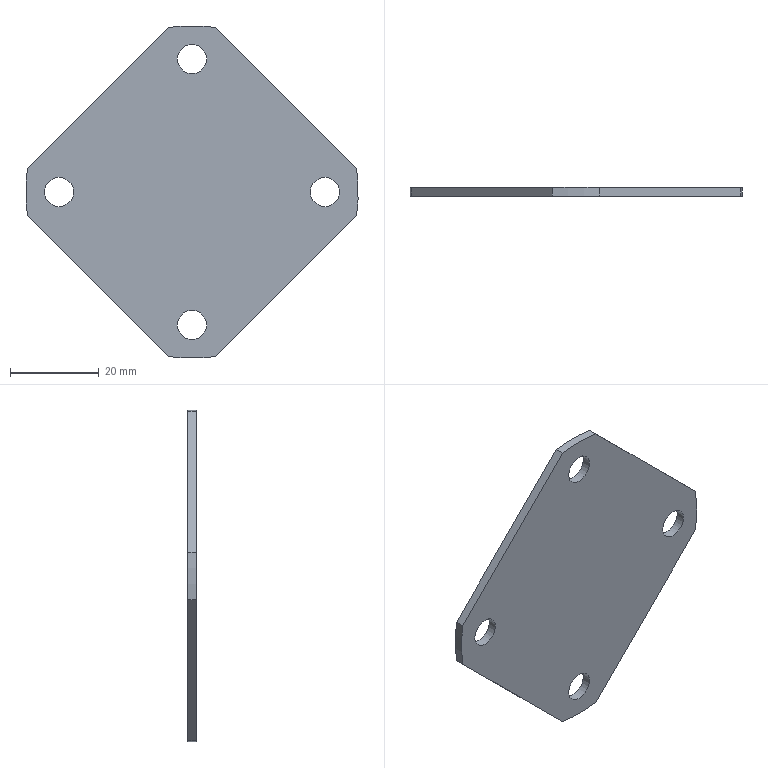Component | NX | DIAPHRAGM | 1 solid | 14 faces | box 75 x 2 x 75 mm | volume 6723 mm3 | cylinder 8 | plane 6 | commonest cylinder face diameters 75 x4 6.6 x4
STEP:
#1=CARTESIAN_POINT('',(0.,0.,0.));
#2=DIRECTION('',(0.,0.,1.));
#3=DIRECTION('',(1.,0.,0.));
#4=AXIS2_PLACEMENT_3D('',#1,#2,#3);
#5=CARTESIAN_POINT('',(-37.123,2.,5.303));
#6=VERTEX_POINT('',#5);
#7=CARTESIAN_POINT('',(-37.123,2.,-5.303));
#8=VERTEX_POINT('',#7);
#9=CARTESIAN_POINT('',(-0.,2.,0.));
#10=DIRECTION('',(0.,-1.,0.));
#11=DIRECTION('',(1.,0.,-0.));
#12=AXIS2_PLACEMENT_3D('',#9,#10,#11);
#13=CIRCLE('',#12,37.5);
#14=CARTESIAN_POINT('',(-0.,0.,0.));
#15=DIRECTION('',(0.,1.,0.));
#16=DIRECTION('',(0.,0.,1.));
#17=AXIS2_PLACEMENT_3D('',#14,#15,#16);
#18=CYLINDRICAL_SURFACE('',#17,37.5);
#19=CARTESIAN_POINT('',(7.854,2.));
#20=DIRECTION('',(-1.,0.));
#21=VECTOR('',#20,1.);
#22=LINE('',#19,#21);
#23=(GEOMETRIC_REPRESENTATION_CONTEXT(2)PARAMETRIC_REPRESENTATION_CONTEXT()REPRESENTATION_CONTEXT('',''));
#24=DEFINITIONAL_REPRESENTATION('',(#22),#23);
#25=PCURVE('',#18,#24);
#26=CARTESIAN_POINT('',(-0.,2.,0.));
#27=DIRECTION('',(0.,-1.,0.));
#28=DIRECTION('',(0.,0.,-1.));
#29=AXIS2_PLACEMENT_3D('',#26,#27,#28);
#30=PLANE('',#29);
#31=CARTESIAN_POINT('',(0.,0.));
#32=DIRECTION('',(0.,1.));
#33=AXIS2_PLACEMENT_2D('',#31,#32);
#34=CIRCLE('',#33,37.5);
#35=(GEOMETRIC_REPRESENTATION_CONTEXT(2)PARAMETRIC_REPRESENTATION_CONTEXT()REPRESENTATION_CONTEXT('',''));
#36=DEFINITIONAL_REPRESENTATION('',(#34),#35);
#37=PCURVE('',#30,#36);
#38=SURFACE_CURVE('',#13,(#25,#37),.PCURVE_S1.);
#39=EDGE_CURVE('',#6,#8,#38,.T.);
#40=ORIENTED_EDGE('',*,*,#39,.T.);
#41=CARTESIAN_POINT('',(-37.123,0.,-5.303));
#42=VERTEX_POINT('',#41);
#43=CARTESIAN_POINT('',(-37.123,0.,-5.303));
#44=DIRECTION('',(0.,1.,0.));
#45=VECTOR('',#44,1.);
#46=LINE('',#43,#45);
#47=CARTESIAN_POINT('',(4.57,0.));
#48=DIRECTION('',(0.,1.));
#49=VECTOR('',#48,1.);
#50=LINE('',#47,#49);
#51=(GEOMETRIC_REPRESENTATION_CONTEXT(2)PARAMETRIC_REPRESENTATION_CONTEXT()REPRESENTATION_CONTEXT('',''));
#52=DEFINITIONAL_REPRESENTATION('',(#50),#51);
#53=PCURVE('',#18,#52);
#54=CARTESIAN_POINT('',(-37.123,0.,-5.303));
#55=DIRECTION('',(0.7071,0.,0.7071));
#56=DIRECTION('',(0.7071,0.,-0.7071));
#57=AXIS2_PLACEMENT_3D('',#54,#55,#56);
#58=PLANE('',#57);
#59=CARTESIAN_POINT('',(0.,0.));
#60=DIRECTION('',(0.,1.));
#61=VECTOR('',#60,1.);
#62=LINE('',#59,#61);
#63=(GEOMETRIC_REPRESENTATION_CONTEXT(2)PARAMETRIC_REPRESENTATION_CONTEXT()REPRESENTATION_CONTEXT('',''));
#64=DEFINITIONAL_REPRESENTATION('',(#62),#63);
#65=PCURVE('',#58,#64);
#66=SURFACE_CURVE('',#46,(#53,#65),.PCURVE_S1.);
#67=EDGE_CURVE('',#42,#8,#66,.T.);
#68=ORIENTED_EDGE('',*,*,#67,.F.);
#69=CARTESIAN_POINT('',(-37.123,0.,5.303));
#70=VERTEX_POINT('',#69);
#71=CARTESIAN_POINT('',(-0.,0.,0.));
#72=DIRECTION('',(0.,-1.,0.));
#73=DIRECTION('',(1.,0.,-0.));
#74=AXIS2_PLACEMENT_3D('',#71,#72,#73);
#75=CIRCLE('',#74,37.5);
#76=CARTESIAN_POINT('',(7.854,0.));
#77=DIRECTION('',(-1.,0.));
#78=VECTOR('',#77,1.);
#79=LINE('',#76,#78);
#80=(GEOMETRIC_REPRESENTATION_CONTEXT(2)PARAMETRIC_REPRESENTATION_CONTEXT()REPRESENTATION_CONTEXT('',''));
#81=DEFINITIONAL_REPRESENTATION('',(#79),#80);
#82=PCURVE('',#18,#81);
#83=CARTESIAN_POINT('',(-0.,0.,0.));
#84=DIRECTION('',(0.,-1.,0.));
#85=DIRECTION('',(0.,0.,-1.));
#86=AXIS2_PLACEMENT_3D('',#83,#84,#85);
#87=PLANE('',#86);
#88=CARTESIAN_POINT('',(0.,0.));
#89=DIRECTION('',(0.,1.));
#90=AXIS2_PLACEMENT_2D('',#88,#89);
#91=CIRCLE('',#90,37.5);
#92=(GEOMETRIC_REPRESENTATION_CONTEXT(2)PARAMETRIC_REPRESENTATION_CONTEXT()REPRESENTATION_CONTEXT('',''));
#93=DEFINITIONAL_REPRESENTATION('',(#91),#92);
#94=PCURVE('',#87,#93);
#95=SURFACE_CURVE('',#75,(#82,#94),.PCURVE_S1.);
#96=EDGE_CURVE('',#70,#42,#95,.T.);
#97=ORIENTED_EDGE('',*,*,#96,.F.);
#98=CARTESIAN_POINT('',(-37.123,0.,5.303));
#99=DIRECTION('',(0.,1.,0.));
#100=VECTOR('',#99,1.);
#101=LINE('',#98,#100);
#102=CARTESIAN_POINT('',(4.854,0.));
#103=DIRECTION('',(0.,1.));
#104=VECTOR('',#103,1.);
#105=LINE('',#102,#104);
#106=(GEOMETRIC_REPRESENTATION_CONTEXT(2)PARAMETRIC_REPRESENTATION_CONTEXT()REPRESENTATION_CONTEXT('',''));
#107=DEFINITIONAL_REPRESENTATION('',(#105),#106);
#108=PCURVE('',#18,#107);
#109=CARTESIAN_POINT('',(-5.303,0.,37.123));
#110=DIRECTION('',(0.7071,0.,-0.7071));
#111=DIRECTION('',(-0.7071,0.,-0.7071));
#112=AXIS2_PLACEMENT_3D('',#109,#110,#111);
#113=PLANE('',#112);
#114=CARTESIAN_POINT('',(45.,0.));
#115=DIRECTION('',(0.,1.));
#116=VECTOR('',#115,1.);
#117=LINE('',#114,#116);
#118=(GEOMETRIC_REPRESENTATION_CONTEXT(2)PARAMETRIC_REPRESENTATION_CONTEXT()REPRESENTATION_CONTEXT('',''));
#119=DEFINITIONAL_REPRESENTATION('',(#117),#118);
#120=PCURVE('',#113,#119);
#121=SURFACE_CURVE('',#101,(#108,#120),.PCURVE_S1.);
#122=EDGE_CURVE('',#70,#6,#121,.T.);
#123=ORIENTED_EDGE('',*,*,#122,.T.);
#124=EDGE_LOOP('',(#40,#68,#97,#123));
#125=FACE_BOUND('',#124,.T.);
#126=ADVANCED_FACE('',(#125),#18,.T.);
#127=CARTESIAN_POINT('',(-5.303,2.,-37.123));
#128=VERTEX_POINT('',#127);
#129=CARTESIAN_POINT('',(-37.123,2.,-5.303));
#130=DIRECTION('',(0.7071,0.,-0.7071));
#131=VECTOR('',#130,1.);
#132=LINE('',#129,#131);
#133=CARTESIAN_POINT('',(0.,2.));
#134=DIRECTION('',(1.,0.));
#135=VECTOR('',#134,1.);
#136=LINE('',#133,#135);
#137=(GEOMETRIC_REPRESENTATION_CONTEXT(2)PARAMETRIC_REPRESENTATION_CONTEXT()REPRESENTATION_CONTEXT('',''));
#138=DEFINITIONAL_REPRESENTATION('',(#136),#137);
#139=PCURVE('',#58,#138);
#140=CARTESIAN_POINT('',(5.303,-37.123));
#141=DIRECTION('',(0.7071,0.7071));
#142=VECTOR('',#141,1.);
#143=LINE('',#140,#142);
#144=(GEOMETRIC_REPRESENTATION_CONTEXT(2)PARAMETRIC_REPRESENTATION_CONTEXT()REPRESENTATION_CONTEXT('',''));
#145=DEFINITIONAL_REPRESENTATION('',(#143),#144);
#146=PCURVE('',#30,#145);
#147=SURFACE_CURVE('',#132,(#139,#146),.PCURVE_S1.);
#148=EDGE_CURVE('',#8,#128,#147,.T.);
#149=ORIENTED_EDGE('',*,*,#148,.T.);
#150=CARTESIAN_POINT('',(-5.303,0.,-37.123));
#151=VERTEX_POINT('',#150);
#152=CARTESIAN_POINT('',(-5.303,0.,-37.123));
#153=DIRECTION('',(0.,1.,0.));
#154=VECTOR('',#153,1.);
#155=LINE('',#152,#154);
#156=CARTESIAN_POINT('',(45.,0.));
#157=DIRECTION('',(0.,1.));
#158=VECTOR('',#157,1.);
#159=LINE('',#156,#158);
#160=(GEOMETRIC_REPRESENTATION_CONTEXT(2)PARAMETRIC_REPRESENTATION_CONTEXT()REPRESENTATION_CONTEXT('',''));
#161=DEFINITIONAL_REPRESENTATION('',(#159),#160);
#162=PCURVE('',#58,#161);
#163=CARTESIAN_POINT('',(-0.,0.,0.));
#164=DIRECTION('',(0.,1.,0.));
#165=DIRECTION('',(0.,0.,1.));
#166=AXIS2_PLACEMENT_3D('',#163,#164,#165);
#167=CYLINDRICAL_SURFACE('',#166,37.5);
#168=CARTESIAN_POINT('',(3.283,0.));
#169=DIRECTION('',(0.,1.));
#170=VECTOR('',#169,1.);
#171=LINE('',#168,#170);
#172=(GEOMETRIC_REPRESENTATION_CONTEXT(2)PARAMETRIC_REPRESENTATION_CONTEXT()REPRESENTATION_CONTEXT('',''));
#173=DEFINITIONAL_REPRESENTATION('',(#171),#172);
#174=PCURVE('',#167,#173);
#175=SURFACE_CURVE('',#155,(#162,#174),.PCURVE_S1.);
#176=EDGE_CURVE('',#151,#128,#175,.T.);
#177=ORIENTED_EDGE('',*,*,#176,.F.);
#178=CARTESIAN_POINT('',(-37.123,0.,-5.303));
#179=DIRECTION('',(0.7071,0.,-0.7071));
#180=VECTOR('',#179,1.);
#181=LINE('',#178,#180);
#182=CARTESIAN_POINT('',(0.,0.));
#183=DIRECTION('',(1.,0.));
#184=VECTOR('',#183,1.);
#185=LINE('',#182,#184);
#186=(GEOMETRIC_REPRESENTATION_CONTEXT(2)PARAMETRIC_REPRESENTATION_CONTEXT()REPRESENTATION_CONTEXT('',''));
#187=DEFINITIONAL_REPRESENTATION('',(#185),#186);
#188=PCURVE('',#58,#187);
#189=CARTESIAN_POINT('',(5.303,-37.123));
#190=DIRECTION('',(0.7071,0.7071));
#191=VECTOR('',#190,1.);
#192=LINE('',#189,#191);
#193=(GEOMETRIC_REPRESENTATION_CONTEXT(2)PARAMETRIC_REPRESENTATION_CONTEXT()REPRESENTATION_CONTEXT('',''));
#194=DEFINITIONAL_REPRESENTATION('',(#192),#193);
#195=PCURVE('',#87,#194);
#196=SURFACE_CURVE('',#181,(#188,#195),.PCURVE_S1.);
#197=EDGE_CURVE('',#42,#151,#196,.T.);
#198=ORIENTED_EDGE('',*,*,#197,.F.);
#199=ORIENTED_EDGE('',*,*,#67,.T.);
#200=EDGE_LOOP('',(#149,#177,#198,#199));
#201=FACE_BOUND('',#200,.T.);
#202=ADVANCED_FACE('',(#201),#58,.F.);
#203=CARTESIAN_POINT('',(5.303,2.,-37.123));
#204=VERTEX_POINT('',#203);
#205=CARTESIAN_POINT('',(-0.,2.,0.));
#206=DIRECTION('',(0.,-1.,0.));
#207=DIRECTION('',(1.,0.,-0.));
#208=AXIS2_PLACEMENT_3D('',#205,#206,#207);
#209=CIRCLE('',#208,37.5);
#210=CARTESIAN_POINT('',(7.854,2.));
#211=DIRECTION('',(-1.,0.));
#212=VECTOR('',#211,1.);
#213=LINE('',#210,#212);
#214=(GEOMETRIC_REPRESENTATION_CONTEXT(2)PARAMETRIC_REPRESENTATION_CONTEXT()REPRESENTATION_CONTEXT('',''));
#215=DEFINITIONAL_REPRESENTATION('',(#213),#214);
#216=PCURVE('',#167,#215);
#217=CARTESIAN_POINT('',(0.,0.));
#218=DIRECTION('',(0.,1.));
#219=AXIS2_PLACEMENT_2D('',#217,#218);
#220=CIRCLE('',#219,37.5);
#221=(GEOMETRIC_REPRESENTATION_CONTEXT(2)PARAMETRIC_REPRESENTATION_CONTEXT()REPRESENTATION_CONTEXT('',''));
#222=DEFINITIONAL_REPRESENTATION('',(#220),#221);
#223=PCURVE('',#30,#222);
#224=SURFACE_CURVE('',#209,(#216,#223),.PCURVE_S1.);
#225=EDGE_CURVE('',#128,#204,#224,.T.);
#226=ORIENTED_EDGE('',*,*,#225,.T.);
#227=CARTESIAN_POINT('',(5.303,0.,-37.123));
#228=VERTEX_POINT('',#227);
#229=CARTESIAN_POINT('',(5.303,0.,-37.123));
#230=DIRECTION('',(0.,1.,0.));
#231=VECTOR('',#230,1.);
#232=LINE('',#229,#231);
#233=CARTESIAN_POINT('',(3.,0.));
#234=DIRECTION('',(0.,1.));
#235=VECTOR('',#234,1.);
#236=LINE('',#233,#235);
#237=(GEOMETRIC_REPRESENTATION_CONTEXT(2)PARAMETRIC_REPRESENTATION_CONTEXT()REPRESENTATION_CONTEXT('',''));
#238=DEFINITIONAL_REPRESENTATION('',(#236),#237);
#239=PCURVE('',#167,#238);
#240=CARTESIAN_POINT('',(5.303,0.,-37.123));
#241=DIRECTION('',(-0.7071,0.,0.7071));
#242=DIRECTION('',(0.7071,0.,0.7071));
#243=AXIS2_PLACEMENT_3D('',#240,#241,#242);
#244=PLANE('',#243);
#245=CARTESIAN_POINT('',(0.,0.));
#246=DIRECTION('',(0.,1.));
#247=VECTOR('',#246,1.);
#248=LINE('',#245,#247);
#249=(GEOMETRIC_REPRESENTATION_CONTEXT(2)PARAMETRIC_REPRESENTATION_CONTEXT()REPRESENTATION_CONTEXT('',''));
#250=DEFINITIONAL_REPRESENTATION('',(#248),#249);
#251=PCURVE('',#244,#250);
#252=SURFACE_CURVE('',#232,(#239,#251),.PCURVE_S1.);
#253=EDGE_CURVE('',#228,#204,#252,.T.);
#254=ORIENTED_EDGE('',*,*,#253,.F.);
#255=CARTESIAN_POINT('',(-0.,0.,0.));
#256=DIRECTION('',(0.,-1.,0.));
#257=DIRECTION('',(1.,0.,-0.));
#258=AXIS2_PLACEMENT_3D('',#255,#256,#257);
#259=CIRCLE('',#258,37.5);
#260=CARTESIAN_POINT('',(7.854,0.));
#261=DIRECTION('',(-1.,0.));
#262=VECTOR('',#261,1.);
#263=LINE('',#260,#262);
#264=(GEOMETRIC_REPRESENTATION_CONTEXT(2)PARAMETRIC_REPRESENTATION_CONTEXT()REPRESENTATION_CONTEXT('',''));
#265=DEFINITIONAL_REPRESENTATION('',(#263),#264);
#266=PCURVE('',#167,#265);
#267=CARTESIAN_POINT('',(0.,0.));
#268=DIRECTION('',(0.,1.));
#269=AXIS2_PLACEMENT_2D('',#267,#268);
#270=CIRCLE('',#269,37.5);
#271=(GEOMETRIC_REPRESENTATION_CONTEXT(2)PARAMETRIC_REPRESENTATION_CONTEXT()REPRESENTATION_CONTEXT('',''));
#272=DEFINITIONAL_REPRESENTATION('',(#270),#271);
#273=PCURVE('',#87,#272);
#274=SURFACE_CURVE('',#259,(#266,#273),.PCURVE_S1.);
#275=EDGE_CURVE('',#151,#228,#274,.T.);
#276=ORIENTED_EDGE('',*,*,#275,.F.);
#277=ORIENTED_EDGE('',*,*,#176,.T.);
#278=EDGE_LOOP('',(#226,#254,#276,#277));
#279=FACE_BOUND('',#278,.T.);
#280=ADVANCED_FACE('',(#279),#167,.T.);
#281=CARTESIAN_POINT('',(37.123,2.,-5.303));
#282=VERTEX_POINT('',#281);
#283=CARTESIAN_POINT('',(5.303,2.,-37.123));
#284=DIRECTION('',(0.7071,0.,0.7071));
#285=VECTOR('',#284,1.);
#286=LINE('',#283,#285);
#287=CARTESIAN_POINT('',(0.,2.));
#288=DIRECTION('',(1.,0.));
#289=VECTOR('',#288,1.);
#290=LINE('',#287,#289);
#291=(GEOMETRIC_REPRESENTATION_CONTEXT(2)PARAMETRIC_REPRESENTATION_CONTEXT()REPRESENTATION_CONTEXT('',''));
#292=DEFINITIONAL_REPRESENTATION('',(#290),#291);
#293=PCURVE('',#244,#292);
#294=CARTESIAN_POINT('',(37.123,5.303));
#295=DIRECTION('',(-0.7071,0.7071));
#296=VECTOR('',#295,1.);
#297=LINE('',#294,#296);
#298=(GEOMETRIC_REPRESENTATION_CONTEXT(2)PARAMETRIC_REPRESENTATION_CONTEXT()REPRESENTATION_CONTEXT('',''));
#299=DEFINITIONAL_REPRESENTATION('',(#297),#298);
#300=PCURVE('',#30,#299);
#301=SURFACE_CURVE('',#286,(#293,#300),.PCURVE_S1.);
#302=EDGE_CURVE('',#204,#282,#301,.T.);
#303=ORIENTED_EDGE('',*,*,#302,.T.);
#304=CARTESIAN_POINT('',(37.123,0.,-5.303));
#305=VERTEX_POINT('',#304);
#306=CARTESIAN_POINT('',(37.123,0.,-5.303));
#307=DIRECTION('',(0.,1.,0.));
#308=VECTOR('',#307,1.);
#309=LINE('',#306,#308);
#310=CARTESIAN_POINT('',(45.,0.));
#311=DIRECTION('',(0.,1.));
#312=VECTOR('',#311,1.);
#313=LINE('',#310,#312);
#314=(GEOMETRIC_REPRESENTATION_CONTEXT(2)PARAMETRIC_REPRESENTATION_CONTEXT()REPRESENTATION_CONTEXT('',''));
#315=DEFINITIONAL_REPRESENTATION('',(#313),#314);
#316=PCURVE('',#244,#315);
#317=CARTESIAN_POINT('',(-0.,0.,0.));
#318=DIRECTION('',(0.,1.,0.));
#319=DIRECTION('',(0.,0.,1.));
#320=AXIS2_PLACEMENT_3D('',#317,#318,#319);
#321=CYLINDRICAL_SURFACE('',#320,37.5);
#322=CARTESIAN_POINT('',(1.713,0.));
#323=DIRECTION('',(0.,1.));
#324=VECTOR('',#323,1.);
#325=LINE('',#322,#324);
#326=(GEOMETRIC_REPRESENTATION_CONTEXT(2)PARAMETRIC_REPRESENTATION_CONTEXT()REPRESENTATION_CONTEXT('',''));
#327=DEFINITIONAL_REPRESENTATION('',(#325),#326);
#328=PCURVE('',#321,#327);
#329=SURFACE_CURVE('',#309,(#316,#328),.PCURVE_S1.);
#330=EDGE_CURVE('',#305,#282,#329,.T.);
#331=ORIENTED_EDGE('',*,*,#330,.F.);
#332=CARTESIAN_POINT('',(5.303,0.,-37.123));
#333=DIRECTION('',(0.7071,0.,0.7071));
#334=VECTOR('',#333,1.);
#335=LINE('',#332,#334);
#336=CARTESIAN_POINT('',(0.,0.));
#337=DIRECTION('',(1.,0.));
#338=VECTOR('',#337,1.);
#339=LINE('',#336,#338);
#340=(GEOMETRIC_REPRESENTATION_CONTEXT(2)PARAMETRIC_REPRESENTATION_CONTEXT()REPRESENTATION_CONTEXT('',''));
#341=DEFINITIONAL_REPRESENTATION('',(#339),#340);
#342=PCURVE('',#244,#341);
#343=CARTESIAN_POINT('',(37.123,5.303));
#344=DIRECTION('',(-0.7071,0.7071));
#345=VECTOR('',#344,1.);
#346=LINE('',#343,#345);
#347=(GEOMETRIC_REPRESENTATION_CONTEXT(2)PARAMETRIC_REPRESENTATION_CONTEXT()REPRESENTATION_CONTEXT('',''));
#348=DEFINITIONAL_REPRESENTATION('',(#346),#347);
#349=PCURVE('',#87,#348);
#350=SURFACE_CURVE('',#335,(#342,#349),.PCURVE_S1.);
#351=EDGE_CURVE('',#228,#305,#350,.T.);
#352=ORIENTED_EDGE('',*,*,#351,.F.);
#353=ORIENTED_EDGE('',*,*,#253,.T.);
#354=EDGE_LOOP('',(#303,#331,#352,#353));
#355=FACE_BOUND('',#354,.T.);
#356=ADVANCED_FACE('',(#355),#244,.F.);
#357=CARTESIAN_POINT('',(37.123,2.,5.303));
#358=VERTEX_POINT('',#357);
#359=CARTESIAN_POINT('',(-0.,2.,0.));
#360=DIRECTION('',(0.,-1.,0.));
#361=DIRECTION('',(1.,0.,-0.));
#362=AXIS2_PLACEMENT_3D('',#359,#360,#361);
#363=CIRCLE('',#362,37.5);
#364=CARTESIAN_POINT('',(7.854,2.));
#365=DIRECTION('',(-1.,0.));
#366=VECTOR('',#365,1.);
#367=LINE('',#364,#366);
#368=(GEOMETRIC_REPRESENTATION_CONTEXT(2)PARAMETRIC_REPRESENTATION_CONTEXT()REPRESENTATION_CONTEXT('',''));
#369=DEFINITIONAL_REPRESENTATION('',(#367),#368);
#370=PCURVE('',#321,#369);
#371=CARTESIAN_POINT('',(0.,0.));
#372=DIRECTION('',(0.,1.));
#373=AXIS2_PLACEMENT_2D('',#371,#372);
#374=CIRCLE('',#373,37.5);
#375=(GEOMETRIC_REPRESENTATION_CONTEXT(2)PARAMETRIC_REPRESENTATION_CONTEXT()REPRESENTATION_CONTEXT('',''));
#376=DEFINITIONAL_REPRESENTATION('',(#374),#375);
#377=PCURVE('',#30,#376);
#378=SURFACE_CURVE('',#363,(#370,#377),.PCURVE_S1.);
#379=EDGE_CURVE('',#282,#358,#378,.T.);
#380=ORIENTED_EDGE('',*,*,#379,.T.);
#381=CARTESIAN_POINT('',(37.123,0.,5.303));
#382=VERTEX_POINT('',#381);
#383=CARTESIAN_POINT('',(37.123,0.,5.303));
#384=DIRECTION('',(0.,1.,0.));
#385=VECTOR('',#384,1.);
#386=LINE('',#383,#385);
#387=CARTESIAN_POINT('',(1.429,0.));
#388=DIRECTION('',(0.,1.));
#389=VECTOR('',#388,1.);
#390=LINE('',#387,#389);
#391=(GEOMETRIC_REPRESENTATION_CONTEXT(2)PARAMETRIC_REPRESENTATION_CONTEXT()REPRESENTATION_CONTEXT('',''));
#392=DEFINITIONAL_REPRESENTATION('',(#390),#391);
#393=PCURVE('',#321,#392);
#394=CARTESIAN_POINT('',(37.123,0.,5.303));
#395=DIRECTION('',(-0.7071,0.,-0.7071));
#396=DIRECTION('',(-0.7071,0.,0.7071));
#397=AXIS2_PLACEMENT_3D('',#394,#395,#396);
#398=PLANE('',#397);
#399=CARTESIAN_POINT('',(0.,0.));
#400=DIRECTION('',(0.,1.));
#401=VECTOR('',#400,1.);
#402=LINE('',#399,#401);
#403=(GEOMETRIC_REPRESENTATION_CONTEXT(2)PARAMETRIC_REPRESENTATION_CONTEXT()REPRESENTATION_CONTEXT('',''));
#404=DEFINITIONAL_REPRESENTATION('',(#402),#403);
#405=PCURVE('',#398,#404);
#406=SURFACE_CURVE('',#386,(#393,#405),.PCURVE_S1.);
#407=EDGE_CURVE('',#382,#358,#406,.T.);
#408=ORIENTED_EDGE('',*,*,#407,.F.);
#409=CARTESIAN_POINT('',(-0.,0.,0.));
#410=DIRECTION('',(0.,-1.,0.));
#411=DIRECTION('',(1.,0.,-0.));
#412=AXIS2_PLACEMENT_3D('',#409,#410,#411);
#413=CIRCLE('',#412,37.5);
#414=CARTESIAN_POINT('',(7.854,0.));
#415=DIRECTION('',(-1.,0.));
#416=VECTOR('',#415,1.);
#417=LINE('',#414,#416);
#418=(GEOMETRIC_REPRESENTATION_CONTEXT(2)PARAMETRIC_REPRESENTATION_CONTEXT()REPRESENTATION_CONTEXT('',''));
#419=DEFINITIONAL_REPRESENTATION('',(#417),#418);
#420=PCURVE('',#321,#419);
#421=CARTESIAN_POINT('',(0.,0.));
#422=DIRECTION('',(0.,1.));
#423=AXIS2_PLACEMENT_2D('',#421,#422);
#424=CIRCLE('',#423,37.5);
#425=(GEOMETRIC_REPRESENTATION_CONTEXT(2)PARAMETRIC_REPRESENTATION_CONTEXT()REPRESENTATION_CONTEXT('',''));
#426=DEFINITIONAL_REPRESENTATION('',(#424),#425);
#427=PCURVE('',#87,#426);
#428=SURFACE_CURVE('',#413,(#420,#427),.PCURVE_S1.);
#429=EDGE_CURVE('',#305,#382,#428,.T.);
#430=ORIENTED_EDGE('',*,*,#429,.F.);
#431=ORIENTED_EDGE('',*,*,#330,.T.);
#432=EDGE_LOOP('',(#380,#408,#430,#431));
#433=FACE_BOUND('',#432,.T.);
#434=ADVANCED_FACE('',(#433),#321,.T.);
#435=CARTESIAN_POINT('',(5.303,2.,37.123));
#436=VERTEX_POINT('',#435);
#437=CARTESIAN_POINT('',(37.123,2.,5.303));
#438=DIRECTION('',(-0.7071,0.,0.7071));
#439=VECTOR('',#438,1.);
#440=LINE('',#437,#439);
#441=CARTESIAN_POINT('',(0.,2.));
#442=DIRECTION('',(1.,0.));
#443=VECTOR('',#442,1.);
#444=LINE('',#441,#443);
#445=(GEOMETRIC_REPRESENTATION_CONTEXT(2)PARAMETRIC_REPRESENTATION_CONTEXT()REPRESENTATION_CONTEXT('',''));
#446=DEFINITIONAL_REPRESENTATION('',(#444),#445);
#447=PCURVE('',#398,#446);
#448=CARTESIAN_POINT('',(-5.303,37.123));
#449=DIRECTION('',(-0.7071,-0.7071));
#450=VECTOR('',#449,1.);
#451=LINE('',#448,#450);
#452=(GEOMETRIC_REPRESENTATION_CONTEXT(2)PARAMETRIC_REPRESENTATION_CONTEXT()REPRESENTATION_CONTEXT('',''));
#453=DEFINITIONAL_REPRESENTATION('',(#451),#452);
#454=PCURVE('',#30,#453);
#455=SURFACE_CURVE('',#440,(#447,#454),.PCURVE_S1.);
#456=EDGE_CURVE('',#358,#436,#455,.T.);
#457=ORIENTED_EDGE('',*,*,#456,.T.);
#458=CARTESIAN_POINT('',(5.303,0.,37.123));
#459=VERTEX_POINT('',#458);
#460=CARTESIAN_POINT('',(5.303,0.,37.123));
#461=DIRECTION('',(0.,1.,0.));
#462=VECTOR('',#461,1.);
#463=LINE('',#460,#462);
#464=CARTESIAN_POINT('',(45.,0.));
#465=DIRECTION('',(0.,1.));
#466=VECTOR('',#465,1.);
#467=LINE('',#464,#466);
#468=(GEOMETRIC_REPRESENTATION_CONTEXT(2)PARAMETRIC_REPRESENTATION_CONTEXT()REPRESENTATION_CONTEXT('',''));
#469=DEFINITIONAL_REPRESENTATION('',(#467),#468);
#470=PCURVE('',#398,#469);
#471=CARTESIAN_POINT('',(-0.,0.,0.));
#472=DIRECTION('',(0.,1.,0.));
#473=DIRECTION('',(0.,0.,1.));
#474=AXIS2_PLACEMENT_3D('',#471,#472,#473);
#475=CYLINDRICAL_SURFACE('',#474,37.5);
#476=CARTESIAN_POINT('',(0.1419,0.));
#477=DIRECTION('',(0.,1.));
#478=VECTOR('',#477,1.);
#479=LINE('',#476,#478);
#480=(GEOMETRIC_REPRESENTATION_CONTEXT(2)PARAMETRIC_REPRESENTATION_CONTEXT()REPRESENTATION_CONTEXT('',''));
#481=DEFINITIONAL_REPRESENTATION('',(#479),#480);
#482=PCURVE('',#475,#481);
#483=SURFACE_CURVE('',#463,(#470,#482),.PCURVE_S1.);
#484=EDGE_CURVE('',#459,#436,#483,.T.);
#485=ORIENTED_EDGE('',*,*,#484,.F.);
#486=CARTESIAN_POINT('',(37.123,0.,5.303));
#487=DIRECTION('',(-0.7071,0.,0.7071));
#488=VECTOR('',#487,1.);
#489=LINE('',#486,#488);
#490=CARTESIAN_POINT('',(0.,0.));
#491=DIRECTION('',(1.,0.));
#492=VECTOR('',#491,1.);
#493=LINE('',#490,#492);
#494=(GEOMETRIC_REPRESENTATION_CONTEXT(2)PARAMETRIC_REPRESENTATION_CONTEXT()REPRESENTATION_CONTEXT('',''));
#495=DEFINITIONAL_REPRESENTATION('',(#493),#494);
#496=PCURVE('',#398,#495);
#497=CARTESIAN_POINT('',(-5.303,37.123));
#498=DIRECTION('',(-0.7071,-0.7071));
#499=VECTOR('',#498,1.);
#500=LINE('',#497,#499);
#501=(GEOMETRIC_REPRESENTATION_CONTEXT(2)PARAMETRIC_REPRESENTATION_CONTEXT()REPRESENTATION_CONTEXT('',''));
#502=DEFINITIONAL_REPRESENTATION('',(#500),#501);
#503=PCURVE('',#87,#502);
#504=SURFACE_CURVE('',#489,(#496,#503),.PCURVE_S1.);
#505=EDGE_CURVE('',#382,#459,#504,.T.);
#506=ORIENTED_EDGE('',*,*,#505,.F.);
#507=ORIENTED_EDGE('',*,*,#407,.T.);
#508=EDGE_LOOP('',(#457,#485,#506,#507));
#509=FACE_BOUND('',#508,.T.);
#510=ADVANCED_FACE('',(#509),#398,.F.);
#511=CARTESIAN_POINT('',(-5.303,2.,37.123));
#512=VERTEX_POINT('',#511);
#513=CARTESIAN_POINT('',(-0.,2.,0.));
#514=DIRECTION('',(0.,-1.,0.));
#515=DIRECTION('',(1.,0.,-0.));
#516=AXIS2_PLACEMENT_3D('',#513,#514,#515);
#517=CIRCLE('',#516,37.5);
#518=CARTESIAN_POINT('',(1.571,2.));
#519=DIRECTION('',(-1.,0.));
#520=VECTOR('',#519,1.);
#521=LINE('',#518,#520);
#522=(GEOMETRIC_REPRESENTATION_CONTEXT(2)PARAMETRIC_REPRESENTATION_CONTEXT()REPRESENTATION_CONTEXT('',''));
#523=DEFINITIONAL_REPRESENTATION('',(#521),#522);
#524=PCURVE('',#475,#523);
#525=CARTESIAN_POINT('',(0.,0.));
#526=DIRECTION('',(0.,1.));
#527=AXIS2_PLACEMENT_2D('',#525,#526);
#528=CIRCLE('',#527,37.5);
#529=(GEOMETRIC_REPRESENTATION_CONTEXT(2)PARAMETRIC_REPRESENTATION_CONTEXT()REPRESENTATION_CONTEXT('',''));
#530=DEFINITIONAL_REPRESENTATION('',(#528),#529);
#531=PCURVE('',#30,#530);
#532=SURFACE_CURVE('',#517,(#524,#531),.PCURVE_S1.);
#533=EDGE_CURVE('',#436,#512,#532,.T.);
#534=ORIENTED_EDGE('',*,*,#533,.T.);
#535=CARTESIAN_POINT('',(-5.303,0.,37.123));
#536=VERTEX_POINT('',#535);
#537=CARTESIAN_POINT('',(-5.303,0.,37.123));
#538=DIRECTION('',(0.,1.,0.));
#539=VECTOR('',#538,1.);
#540=LINE('',#537,#539);
#541=CARTESIAN_POINT('',(-0.1419,0.));
#542=DIRECTION('',(0.,1.));
#543=VECTOR('',#542,1.);
#544=LINE('',#541,#543);
#545=(GEOMETRIC_REPRESENTATION_CONTEXT(2)PARAMETRIC_REPRESENTATION_CONTEXT()REPRESENTATION_CONTEXT('',''));
#546=DEFINITIONAL_REPRESENTATION('',(#544),#545);
#547=PCURVE('',#475,#546);
#548=CARTESIAN_POINT('',(-0.,0.));
#549=DIRECTION('',(0.,1.));
#550=VECTOR('',#549,1.);
#551=LINE('',#548,#550);
#552=(GEOMETRIC_REPRESENTATION_CONTEXT(2)PARAMETRIC_REPRESENTATION_CONTEXT()REPRESENTATION_CONTEXT('',''));
#553=DEFINITIONAL_REPRESENTATION('',(#551),#552);
#554=PCURVE('',#113,#553);
#555=SURFACE_CURVE('',#540,(#547,#554),.PCURVE_S1.);
#556=EDGE_CURVE('',#536,#512,#555,.T.);
#557=ORIENTED_EDGE('',*,*,#556,.F.);
#558=CARTESIAN_POINT('',(-0.,0.,0.));
#559=DIRECTION('',(0.,-1.,0.));
#560=DIRECTION('',(1.,0.,-0.));
#561=AXIS2_PLACEMENT_3D('',#558,#559,#560);
#562=CIRCLE('',#561,37.5);
#563=CARTESIAN_POINT('',(1.571,0.));
#564=DIRECTION('',(-1.,0.));
#565=VECTOR('',#564,1.);
#566=LINE('',#563,#565);
#567=(GEOMETRIC_REPRESENTATION_CONTEXT(2)PARAMETRIC_REPRESENTATION_CONTEXT()REPRESENTATION_CONTEXT('',''));
#568=DEFINITIONAL_REPRESENTATION('',(#566),#567);
#569=PCURVE('',#475,#568);
#570=CARTESIAN_POINT('',(0.,0.));
#571=DIRECTION('',(0.,1.));
#572=AXIS2_PLACEMENT_2D('',#570,#571);
#573=CIRCLE('',#572,37.5);
#574=(GEOMETRIC_REPRESENTATION_CONTEXT(2)PARAMETRIC_REPRESENTATION_CONTEXT()REPRESENTATION_CONTEXT('',''));
#575=DEFINITIONAL_REPRESENTATION('',(#573),#574);
#576=PCURVE('',#87,#575);
#577=SURFACE_CURVE('',#562,(#569,#576),.PCURVE_S1.);
#578=EDGE_CURVE('',#459,#536,#577,.T.);
#579=ORIENTED_EDGE('',*,*,#578,.F.);
#580=ORIENTED_EDGE('',*,*,#484,.T.);
#581=EDGE_LOOP('',(#534,#557,#579,#580));
#582=FACE_BOUND('',#581,.T.);
#583=ADVANCED_FACE('',(#582),#475,.T.);
#584=CARTESIAN_POINT('',(-3.3,0.,-30.));
#585=VERTEX_POINT('',#584);
#586=CARTESIAN_POINT('',(-0.,0.,-30.));
#587=DIRECTION('',(0.,-1.,0.));
#588=DIRECTION('',(-1.,0.,0.));
#589=AXIS2_PLACEMENT_3D('',#586,#587,#588);
#590=CIRCLE('',#589,3.3);
#591=CARTESIAN_POINT('',(-0.,0.,-30.));
#592=DIRECTION('',(0.,1.,0.));
#593=DIRECTION('',(0.,0.,1.));
#594=AXIS2_PLACEMENT_3D('',#591,#592,#593);
#595=CYLINDRICAL_SURFACE('',#594,3.3);
#596=CARTESIAN_POINT('',(10.996,0.));
#597=DIRECTION('',(-1.,0.));
#598=VECTOR('',#597,1.);
#599=LINE('',#596,#598);
#600=(GEOMETRIC_REPRESENTATION_CONTEXT(2)PARAMETRIC_REPRESENTATION_CONTEXT()REPRESENTATION_CONTEXT('',''));
#601=DEFINITIONAL_REPRESENTATION('',(#599),#600);
#602=PCURVE('',#595,#601);
#603=CARTESIAN_POINT('',(30.,0.));
#604=DIRECTION('',(0.,-1.));
#605=AXIS2_PLACEMENT_2D('',#603,#604);
#606=CIRCLE('',#605,3.3);
#607=(GEOMETRIC_REPRESENTATION_CONTEXT(2)PARAMETRIC_REPRESENTATION_CONTEXT()REPRESENTATION_CONTEXT('',''));
#608=DEFINITIONAL_REPRESENTATION('',(#606),#607);
#609=PCURVE('',#87,#608);
#610=SURFACE_CURVE('',#590,(#602,#609),.PCURVE_S1.);
#611=EDGE_CURVE('',#585,#585,#610,.T.);
#612=ORIENTED_EDGE('',*,*,#611,.F.);
#613=CARTESIAN_POINT('',(-3.3,2.,-30.));
#614=VERTEX_POINT('',#613);
#615=CARTESIAN_POINT('',(-3.3,0.,-30.));
#616=CARTESIAN_POINT('',(-3.3,2.,-30.));
#617=B_SPLINE_CURVE_WITH_KNOTS('',1,(#615,#616),.UNSPECIFIED.,.F.,.F.,(2,2),(0.,2.),.PIECEWISE_BEZIER_KNOTS.);
#618=CARTESIAN_POINT('',(10.996,0.));
#619=DIRECTION('',(0.,1.));
#620=VECTOR('',#619,1.);
#621=LINE('',#618,#620);
#622=(GEOMETRIC_REPRESENTATION_CONTEXT(2)PARAMETRIC_REPRESENTATION_CONTEXT()REPRESENTATION_CONTEXT('',''));
#623=DEFINITIONAL_REPRESENTATION('',(#621),#622);
#624=PCURVE('',#595,#623);
#625=CARTESIAN_POINT('',(4.712,0.));
#626=DIRECTION('',(0.,1.));
#627=VECTOR('',#626,1.);
#628=LINE('',#625,#627);
#629=(GEOMETRIC_REPRESENTATION_CONTEXT(2)PARAMETRIC_REPRESENTATION_CONTEXT()REPRESENTATION_CONTEXT('',''));
#630=DEFINITIONAL_REPRESENTATION('',(#628),#629);
#631=PCURVE('',#595,#630);
#632=SEAM_CURVE('',#617,(#624,#631),.PCURVE_S1.);
#633=EDGE_CURVE('',#585,#614,#632,.T.);
#634=ORIENTED_EDGE('',*,*,#633,.T.);
#635=CARTESIAN_POINT('',(-0.,2.,-30.));
#636=DIRECTION('',(0.,-1.,0.));
#637=DIRECTION('',(-1.,0.,0.));
#638=AXIS2_PLACEMENT_3D('',#635,#636,#637);
#639=CIRCLE('',#638,3.3);
#640=CARTESIAN_POINT('',(10.996,2.));
#641=DIRECTION('',(-1.,0.));
#642=VECTOR('',#641,1.);
#643=LINE('',#640,#642);
#644=(GEOMETRIC_REPRESENTATION_CONTEXT(2)PARAMETRIC_REPRESENTATION_CONTEXT()REPRESENTATION_CONTEXT('',''));
#645=DEFINITIONAL_REPRESENTATION('',(#643),#644);
#646=PCURVE('',#595,#645);
#647=CARTESIAN_POINT('',(30.,0.));
#648=DIRECTION('',(0.,-1.));
#649=AXIS2_PLACEMENT_2D('',#647,#648);
#650=CIRCLE('',#649,3.3);
#651=(GEOMETRIC_REPRESENTATION_CONTEXT(2)PARAMETRIC_REPRESENTATION_CONTEXT()REPRESENTATION_CONTEXT('',''));
#652=DEFINITIONAL_REPRESENTATION('',(#650),#651);
#653=PCURVE('',#30,#652);
#654=SURFACE_CURVE('',#639,(#646,#653),.PCURVE_S1.);
#655=EDGE_CURVE('',#614,#614,#654,.T.);
#656=ORIENTED_EDGE('',*,*,#655,.T.);
#657=ORIENTED_EDGE('',*,*,#633,.F.);
#658=EDGE_LOOP('',(#612,#634,#656,#657));
#659=FACE_BOUND('',#658,.F.);
#660=ADVANCED_FACE('',(#659),#595,.F.);
#661=CARTESIAN_POINT('',(-30.,0.,3.3));
#662=VERTEX_POINT('',#661);
#663=CARTESIAN_POINT('',(-30.,0.,0.));
#664=DIRECTION('',(0.,-1.,0.));
#665=DIRECTION('',(0.,0.,1.));
#666=AXIS2_PLACEMENT_3D('',#663,#664,#665);
#667=CIRCLE('',#666,3.3);
#668=CARTESIAN_POINT('',(-30.,0.,0.));
#669=DIRECTION('',(0.,1.,0.));
#670=DIRECTION('',(0.,0.,1.));
#671=AXIS2_PLACEMENT_3D('',#668,#669,#670);
#672=CYLINDRICAL_SURFACE('',#671,3.3);
#673=CARTESIAN_POINT('',(6.283,0.));
#674=DIRECTION('',(-1.,0.));
#675=VECTOR('',#674,1.);
#676=LINE('',#673,#675);
#677=(GEOMETRIC_REPRESENTATION_CONTEXT(2)PARAMETRIC_REPRESENTATION_CONTEXT()REPRESENTATION_CONTEXT('',''));
#678=DEFINITIONAL_REPRESENTATION('',(#676),#677);
#679=PCURVE('',#672,#678);
#680=CARTESIAN_POINT('',(0.,-30.));
#681=DIRECTION('',(-1.,0.));
#682=AXIS2_PLACEMENT_2D('',#680,#681);
#683=CIRCLE('',#682,3.3);
#684=(GEOMETRIC_REPRESENTATION_CONTEXT(2)PARAMETRIC_REPRESENTATION_CONTEXT()REPRESENTATION_CONTEXT('',''));
#685=DEFINITIONAL_REPRESENTATION('',(#683),#684);
#686=PCURVE('',#87,#685);
#687=SURFACE_CURVE('',#667,(#679,#686),.PCURVE_S1.);
#688=EDGE_CURVE('',#662,#662,#687,.T.);
#689=ORIENTED_EDGE('',*,*,#688,.F.);
#690=CARTESIAN_POINT('',(-30.,2.,3.3));
#691=VERTEX_POINT('',#690);
#692=CARTESIAN_POINT('',(-30.,0.,3.3));
#693=CARTESIAN_POINT('',(-30.,2.,3.3));
#694=B_SPLINE_CURVE_WITH_KNOTS('',1,(#692,#693),.UNSPECIFIED.,.F.,.F.,(2,2),(0.,2.),.PIECEWISE_BEZIER_KNOTS.);
#695=CARTESIAN_POINT('',(6.283,0.));
#696=DIRECTION('',(0.,1.));
#697=VECTOR('',#696,1.);
#698=LINE('',#695,#697);
#699=(GEOMETRIC_REPRESENTATION_CONTEXT(2)PARAMETRIC_REPRESENTATION_CONTEXT()REPRESENTATION_CONTEXT('',''));
#700=DEFINITIONAL_REPRESENTATION('',(#698),#699);
#701=PCURVE('',#672,#700);
#702=CARTESIAN_POINT('',(0.,0.));
#703=DIRECTION('',(0.,1.));
#704=VECTOR('',#703,1.);
#705=LINE('',#702,#704);
#706=(GEOMETRIC_REPRESENTATION_CONTEXT(2)PARAMETRIC_REPRESENTATION_CONTEXT()REPRESENTATION_CONTEXT('',''));
#707=DEFINITIONAL_REPRESENTATION('',(#705),#706);
#708=PCURVE('',#672,#707);
#709=SEAM_CURVE('',#694,(#701,#708),.PCURVE_S1.);
#710=EDGE_CURVE('',#662,#691,#709,.T.);
#711=ORIENTED_EDGE('',*,*,#710,.T.);
#712=CARTESIAN_POINT('',(-30.,2.,0.));
#713=DIRECTION('',(0.,-1.,0.));
#714=DIRECTION('',(0.,0.,1.));
#715=AXIS2_PLACEMENT_3D('',#712,#713,#714);
#716=CIRCLE('',#715,3.3);
#717=CARTESIAN_POINT('',(6.283,2.));
#718=DIRECTION('',(-1.,0.));
#719=VECTOR('',#718,1.);
#720=LINE('',#717,#719);
#721=(GEOMETRIC_REPRESENTATION_CONTEXT(2)PARAMETRIC_REPRESENTATION_CONTEXT()REPRESENTATION_CONTEXT('',''));
#722=DEFINITIONAL_REPRESENTATION('',(#720),#721);
#723=PCURVE('',#672,#722);
#724=CARTESIAN_POINT('',(0.,-30.));
#725=DIRECTION('',(-1.,0.));
#726=AXIS2_PLACEMENT_2D('',#724,#725);
#727=CIRCLE('',#726,3.3);
#728=(GEOMETRIC_REPRESENTATION_CONTEXT(2)PARAMETRIC_REPRESENTATION_CONTEXT()REPRESENTATION_CONTEXT('',''));
#729=DEFINITIONAL_REPRESENTATION('',(#727),#728);
#730=PCURVE('',#30,#729);
#731=SURFACE_CURVE('',#716,(#723,#730),.PCURVE_S1.);
#732=EDGE_CURVE('',#691,#691,#731,.T.);
#733=ORIENTED_EDGE('',*,*,#732,.T.);
#734=ORIENTED_EDGE('',*,*,#710,.F.);
#735=EDGE_LOOP('',(#689,#711,#733,#734));
#736=FACE_BOUND('',#735,.F.);
#737=ADVANCED_FACE('',(#736),#672,.F.);
#738=CARTESIAN_POINT('',(3.3,0.,30.));
#739=VERTEX_POINT('',#738);
#740=CARTESIAN_POINT('',(-0.,0.,30.));
#741=DIRECTION('',(0.,-1.,0.));
#742=DIRECTION('',(1.,0.,0.));
#743=AXIS2_PLACEMENT_3D('',#740,#741,#742);
#744=CIRCLE('',#743,3.3);
#745=CARTESIAN_POINT('',(-0.,0.,30.));
#746=DIRECTION('',(0.,1.,0.));
#747=DIRECTION('',(0.,0.,1.));
#748=AXIS2_PLACEMENT_3D('',#745,#746,#747);
#749=CYLINDRICAL_SURFACE('',#748,3.3);
#750=CARTESIAN_POINT('',(7.854,0.));
#751=DIRECTION('',(-1.,0.));
#752=VECTOR('',#751,1.);
#753=LINE('',#750,#752);
#754=(GEOMETRIC_REPRESENTATION_CONTEXT(2)PARAMETRIC_REPRESENTATION_CONTEXT()REPRESENTATION_CONTEXT('',''));
#755=DEFINITIONAL_REPRESENTATION('',(#753),#754);
#756=PCURVE('',#749,#755);
#757=CARTESIAN_POINT('',(-30.,0.));
#758=DIRECTION('',(0.,1.));
#759=AXIS2_PLACEMENT_2D('',#757,#758);
#760=CIRCLE('',#759,3.3);
#761=(GEOMETRIC_REPRESENTATION_CONTEXT(2)PARAMETRIC_REPRESENTATION_CONTEXT()REPRESENTATION_CONTEXT('',''));
#762=DEFINITIONAL_REPRESENTATION('',(#760),#761);
#763=PCURVE('',#87,#762);
#764=SURFACE_CURVE('',#744,(#756,#763),.PCURVE_S1.);
#765=EDGE_CURVE('',#739,#739,#764,.T.);
#766=ORIENTED_EDGE('',*,*,#765,.F.);
#767=CARTESIAN_POINT('',(3.3,2.,30.));
#768=VERTEX_POINT('',#767);
#769=CARTESIAN_POINT('',(3.3,0.,30.));
#770=CARTESIAN_POINT('',(3.3,2.,30.));
#771=B_SPLINE_CURVE_WITH_KNOTS('',1,(#769,#770),.UNSPECIFIED.,.F.,.F.,(2,2),(0.,2.),.PIECEWISE_BEZIER_KNOTS.);
#772=CARTESIAN_POINT('',(7.854,0.));
#773=DIRECTION('',(0.,1.));
#774=VECTOR('',#773,1.);
#775=LINE('',#772,#774);
#776=(GEOMETRIC_REPRESENTATION_CONTEXT(2)PARAMETRIC_REPRESENTATION_CONTEXT()REPRESENTATION_CONTEXT('',''));
#777=DEFINITIONAL_REPRESENTATION('',(#775),#776);
#778=PCURVE('',#749,#777);
#779=CARTESIAN_POINT('',(1.571,0.));
#780=DIRECTION('',(0.,1.));
#781=VECTOR('',#780,1.);
#782=LINE('',#779,#781);
#783=(GEOMETRIC_REPRESENTATION_CONTEXT(2)PARAMETRIC_REPRESENTATION_CONTEXT()REPRESENTATION_CONTEXT('',''));
#784=DEFINITIONAL_REPRESENTATION('',(#782),#783);
#785=PCURVE('',#749,#784);
#786=SEAM_CURVE('',#771,(#778,#785),.PCURVE_S1.);
#787=EDGE_CURVE('',#739,#768,#786,.T.);
#788=ORIENTED_EDGE('',*,*,#787,.T.);
#789=CARTESIAN_POINT('',(-0.,2.,30.));
#790=DIRECTION('',(0.,-1.,0.));
#791=DIRECTION('',(1.,0.,0.));
#792=AXIS2_PLACEMENT_3D('',#789,#790,#791);
#793=CIRCLE('',#792,3.3);
#794=CARTESIAN_POINT('',(7.854,2.));
#795=DIRECTION('',(-1.,0.));
#796=VECTOR('',#795,1.);
#797=LINE('',#794,#796);
#798=(GEOMETRIC_REPRESENTATION_CONTEXT(2)PARAMETRIC_REPRESENTATION_CONTEXT()REPRESENTATION_CONTEXT('',''));
#799=DEFINITIONAL_REPRESENTATION('',(#797),#798);
#800=PCURVE('',#749,#799);
#801=CARTESIAN_POINT('',(-30.,0.));
#802=DIRECTION('',(0.,1.));
#803=AXIS2_PLACEMENT_2D('',#801,#802);
#804=CIRCLE('',#803,3.3);
#805=(GEOMETRIC_REPRESENTATION_CONTEXT(2)PARAMETRIC_REPRESENTATION_CONTEXT()REPRESENTATION_CONTEXT('',''));
#806=DEFINITIONAL_REPRESENTATION('',(#804),#805);
#807=PCURVE('',#30,#806);
#808=SURFACE_CURVE('',#793,(#800,#807),.PCURVE_S1.);
#809=EDGE_CURVE('',#768,#768,#808,.T.);
#810=ORIENTED_EDGE('',*,*,#809,.T.);
#811=ORIENTED_EDGE('',*,*,#787,.F.);
#812=EDGE_LOOP('',(#766,#788,#810,#811));
#813=FACE_BOUND('',#812,.F.);
#814=ADVANCED_FACE('',(#813),#749,.F.);
#815=CARTESIAN_POINT('',(-5.303,2.,37.123));
#816=DIRECTION('',(-0.7071,0.,-0.7071));
#817=VECTOR('',#816,1.);
#818=LINE('',#815,#817);
#819=CARTESIAN_POINT('',(0.,2.));
#820=DIRECTION('',(1.,0.));
#821=VECTOR('',#820,1.);
#822=LINE('',#819,#821);
#823=(GEOMETRIC_REPRESENTATION_CONTEXT(2)PARAMETRIC_REPRESENTATION_CONTEXT()REPRESENTATION_CONTEXT('',''));
#824=DEFINITIONAL_REPRESENTATION('',(#822),#823);
#825=PCURVE('',#113,#824);
#826=CARTESIAN_POINT('',(-37.123,-5.303));
#827=DIRECTION('',(0.7071,-0.7071));
#828=VECTOR('',#827,1.);
#829=LINE('',#826,#828);
#830=(GEOMETRIC_REPRESENTATION_CONTEXT(2)PARAMETRIC_REPRESENTATION_CONTEXT()REPRESENTATION_CONTEXT('',''));
#831=DEFINITIONAL_REPRESENTATION('',(#829),#830);
#832=PCURVE('',#30,#831);
#833=SURFACE_CURVE('',#818,(#825,#832),.PCURVE_S1.);
#834=EDGE_CURVE('',#512,#6,#833,.T.);
#835=ORIENTED_EDGE('',*,*,#834,.T.);
#836=ORIENTED_EDGE('',*,*,#122,.F.);
#837=CARTESIAN_POINT('',(-5.303,0.,37.123));
#838=DIRECTION('',(-0.7071,0.,-0.7071));
#839=VECTOR('',#838,1.);
#840=LINE('',#837,#839);
#841=CARTESIAN_POINT('',(0.,0.));
#842=DIRECTION('',(1.,0.));
#843=VECTOR('',#842,1.);
#844=LINE('',#841,#843);
#845=(GEOMETRIC_REPRESENTATION_CONTEXT(2)PARAMETRIC_REPRESENTATION_CONTEXT()REPRESENTATION_CONTEXT('',''));
#846=DEFINITIONAL_REPRESENTATION('',(#844),#845);
#847=PCURVE('',#113,#846);
#848=CARTESIAN_POINT('',(-37.123,-5.303));
#849=DIRECTION('',(0.7071,-0.7071));
#850=VECTOR('',#849,1.);
#851=LINE('',#848,#850);
#852=(GEOMETRIC_REPRESENTATION_CONTEXT(2)PARAMETRIC_REPRESENTATION_CONTEXT()REPRESENTATION_CONTEXT('',''));
#853=DEFINITIONAL_REPRESENTATION('',(#851),#852);
#854=PCURVE('',#87,#853);
#855=SURFACE_CURVE('',#840,(#847,#854),.PCURVE_S1.);
#856=EDGE_CURVE('',#536,#70,#855,.T.);
#857=ORIENTED_EDGE('',*,*,#856,.F.);
#858=ORIENTED_EDGE('',*,*,#556,.T.);
#859=EDGE_LOOP('',(#835,#836,#857,#858));
#860=FACE_BOUND('',#859,.T.);
#861=ADVANCED_FACE('',(#860),#113,.F.);
#862=CARTESIAN_POINT('',(30.,0.,-3.3));
#863=VERTEX_POINT('',#862);
#864=CARTESIAN_POINT('',(30.,0.,0.));
#865=DIRECTION('',(0.,-1.,0.));
#866=DIRECTION('',(0.,0.,-1.));
#867=AXIS2_PLACEMENT_3D('',#864,#865,#866);
#868=CIRCLE('',#867,3.3);
#869=CARTESIAN_POINT('',(30.,0.,0.));
#870=DIRECTION('',(0.,1.,0.));
#871=DIRECTION('',(0.,0.,1.));
#872=AXIS2_PLACEMENT_3D('',#869,#870,#871);
#873=CYLINDRICAL_SURFACE('',#872,3.3);
#874=CARTESIAN_POINT('',(9.425,0.));
#875=DIRECTION('',(-1.,0.));
#876=VECTOR('',#875,1.);
#877=LINE('',#874,#876);
#878=(GEOMETRIC_REPRESENTATION_CONTEXT(2)PARAMETRIC_REPRESENTATION_CONTEXT()REPRESENTATION_CONTEXT('',''));
#879=DEFINITIONAL_REPRESENTATION('',(#877),#878);
#880=PCURVE('',#873,#879);
#881=CARTESIAN_POINT('',(0.,30.));
#882=DIRECTION('',(1.,0.));
#883=AXIS2_PLACEMENT_2D('',#881,#882);
#884=CIRCLE('',#883,3.3);
#885=(GEOMETRIC_REPRESENTATION_CONTEXT(2)PARAMETRIC_REPRESENTATION_CONTEXT()REPRESENTATION_CONTEXT('',''));
#886=DEFINITIONAL_REPRESENTATION('',(#884),#885);
#887=PCURVE('',#87,#886);
#888=SURFACE_CURVE('',#868,(#880,#887),.PCURVE_S1.);
#889=EDGE_CURVE('',#863,#863,#888,.T.);
#890=ORIENTED_EDGE('',*,*,#889,.F.);
#891=CARTESIAN_POINT('',(30.,2.,-3.3));
#892=VERTEX_POINT('',#891);
#893=CARTESIAN_POINT('',(30.,0.,-3.3));
#894=CARTESIAN_POINT('',(30.,2.,-3.3));
#895=B_SPLINE_CURVE_WITH_KNOTS('',1,(#893,#894),.UNSPECIFIED.,.F.,.F.,(2,2),(0.,2.),.PIECEWISE_BEZIER_KNOTS.);
#896=CARTESIAN_POINT('',(9.425,0.));
#897=DIRECTION('',(0.,1.));
#898=VECTOR('',#897,1.);
#899=LINE('',#896,#898);
#900=(GEOMETRIC_REPRESENTATION_CONTEXT(2)PARAMETRIC_REPRESENTATION_CONTEXT()REPRESENTATION_CONTEXT('',''));
#901=DEFINITIONAL_REPRESENTATION('',(#899),#900);
#902=PCURVE('',#873,#901);
#903=CARTESIAN_POINT('',(3.142,0.));
#904=DIRECTION('',(0.,1.));
#905=VECTOR('',#904,1.);
#906=LINE('',#903,#905);
#907=(GEOMETRIC_REPRESENTATION_CONTEXT(2)PARAMETRIC_REPRESENTATION_CONTEXT()REPRESENTATION_CONTEXT('',''));
#908=DEFINITIONAL_REPRESENTATION('',(#906),#907);
#909=PCURVE('',#873,#908);
#910=SEAM_CURVE('',#895,(#902,#909),.PCURVE_S1.);
#911=EDGE_CURVE('',#863,#892,#910,.T.);
#912=ORIENTED_EDGE('',*,*,#911,.T.);
#913=CARTESIAN_POINT('',(30.,2.,0.));
#914=DIRECTION('',(0.,-1.,0.));
#915=DIRECTION('',(0.,0.,-1.));
#916=AXIS2_PLACEMENT_3D('',#913,#914,#915);
#917=CIRCLE('',#916,3.3);
#918=CARTESIAN_POINT('',(9.425,2.));
#919=DIRECTION('',(-1.,0.));
#920=VECTOR('',#919,1.);
#921=LINE('',#918,#920);
#922=(GEOMETRIC_REPRESENTATION_CONTEXT(2)PARAMETRIC_REPRESENTATION_CONTEXT()REPRESENTATION_CONTEXT('',''));
#923=DEFINITIONAL_REPRESENTATION('',(#921),#922);
#924=PCURVE('',#873,#923);
#925=CARTESIAN_POINT('',(0.,30.));
#926=DIRECTION('',(1.,0.));
#927=AXIS2_PLACEMENT_2D('',#925,#926);
#928=CIRCLE('',#927,3.3);
#929=(GEOMETRIC_REPRESENTATION_CONTEXT(2)PARAMETRIC_REPRESENTATION_CONTEXT()REPRESENTATION_CONTEXT('',''));
#930=DEFINITIONAL_REPRESENTATION('',(#928),#929);
#931=PCURVE('',#30,#930);
#932=SURFACE_CURVE('',#917,(#924,#931),.PCURVE_S1.);
#933=EDGE_CURVE('',#892,#892,#932,.T.);
#934=ORIENTED_EDGE('',*,*,#933,.T.);
#935=ORIENTED_EDGE('',*,*,#911,.F.);
#936=EDGE_LOOP('',(#890,#912,#934,#935));
#937=FACE_BOUND('',#936,.F.);
#938=ADVANCED_FACE('',(#937),#873,.F.);
#939=ORIENTED_EDGE('',*,*,#96,.T.);
#940=ORIENTED_EDGE('',*,*,#197,.T.);
#941=ORIENTED_EDGE('',*,*,#275,.T.);
#942=ORIENTED_EDGE('',*,*,#351,.T.);
#943=ORIENTED_EDGE('',*,*,#429,.T.);
#944=ORIENTED_EDGE('',*,*,#505,.T.);
#945=ORIENTED_EDGE('',*,*,#578,.T.);
#946=ORIENTED_EDGE('',*,*,#856,.T.);
#947=EDGE_LOOP('',(#939,#940,#941,#942,#943,#944,#945,#946));
#948=FACE_BOUND('',#947,.T.);
#949=ORIENTED_EDGE('',*,*,#765,.F.);
#950=EDGE_LOOP('',(#949));
#951=FACE_BOUND('',#950,.T.);
#952=ORIENTED_EDGE('',*,*,#688,.F.);
#953=EDGE_LOOP('',(#952));
#954=FACE_BOUND('',#953,.T.);
#955=ORIENTED_EDGE('',*,*,#611,.F.);
#956=EDGE_LOOP('',(#955));
#957=FACE_BOUND('',#956,.T.);
#958=ORIENTED_EDGE('',*,*,#889,.F.);
#959=EDGE_LOOP('',(#958));
#960=FACE_BOUND('',#959,.T.);
#961=ADVANCED_FACE('',(#948,#951,#954,#957,#960),#87,.T.);
#962=ORIENTED_EDGE('',*,*,#39,.F.);
#963=ORIENTED_EDGE('',*,*,#834,.F.);
#964=ORIENTED_EDGE('',*,*,#533,.F.);
#965=ORIENTED_EDGE('',*,*,#456,.F.);
#966=ORIENTED_EDGE('',*,*,#379,.F.);
#967=ORIENTED_EDGE('',*,*,#302,.F.);
#968=ORIENTED_EDGE('',*,*,#225,.F.);
#969=ORIENTED_EDGE('',*,*,#148,.F.);
#970=EDGE_LOOP('',(#962,#963,#964,#965,#966,#967,#968,#969));
#971=FACE_BOUND('',#970,.T.);
#972=ORIENTED_EDGE('',*,*,#809,.T.);
#973=EDGE_LOOP('',(#972));
#974=FACE_BOUND('',#973,.T.);
#975=ORIENTED_EDGE('',*,*,#732,.T.);
#976=EDGE_LOOP('',(#975));
#977=FACE_BOUND('',#976,.T.);
#978=ORIENTED_EDGE('',*,*,#655,.T.);
#979=EDGE_LOOP('',(#978));
#980=FACE_BOUND('',#979,.T.);
#981=ORIENTED_EDGE('',*,*,#933,.T.);
#982=EDGE_LOOP('',(#981));
#983=FACE_BOUND('',#982,.T.);
#984=ADVANCED_FACE('',(#971,#974,#977,#980,#983),#30,.F.);
#985=CLOSED_SHELL('',(#126,#202,#280,#356,#434,#510,#583,#660,#737,#814,#861,#938,#961,#984));
#986=MANIFOLD_SOLID_BREP('',#985);
#987=(LENGTH_UNIT()NAMED_UNIT(*)SI_UNIT(.MILLI.,.METRE.));
#988=UNCERTAINTY_MEASURE_WITH_UNIT(LENGTH_MEASURE(0.000002),#987,'','');
#989=(NAMED_UNIT(*)PLANE_ANGLE_UNIT()SI_UNIT($,.RADIAN.));
#990=(NAMED_UNIT(*)SI_UNIT($,.STERADIAN.)SOLID_ANGLE_UNIT());
#991=(GEOMETRIC_REPRESENTATION_CONTEXT(3)GLOBAL_UNCERTAINTY_ASSIGNED_CONTEXT((#988))GLOBAL_UNIT_ASSIGNED_CONTEXT((#987,#989,#990))REPRESENTATION_CONTEXT('',''));
#992=ADVANCED_BREP_SHAPE_REPRESENTATION('',(#4,#986),#991);